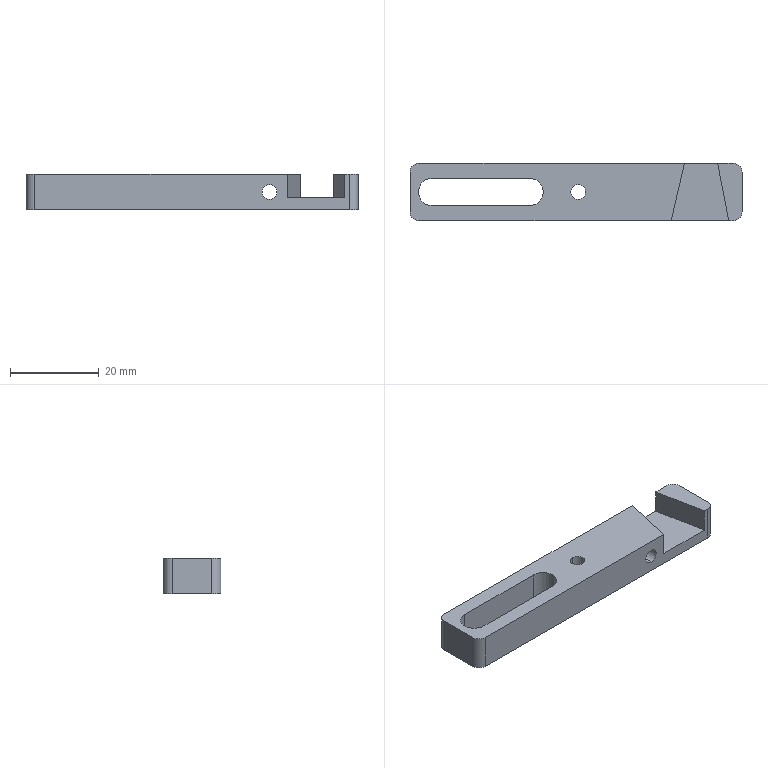Component | SolidWorks | BSH3-02-00ARubberBlankingAssembly2-1_BSH3-02-10FeedBlock2-1 | 1 solid | 22 faces | box 75 x 13 x 8 mm | volume 5554 mm3 | plane 12 | cylinder 10 | commonest cylinder face diameters 3.3 x4 4 x4 6.2 x2
build123d program:
from build123d import *

# Parameters (mm, degrees)
SKETCH1_W         = 13
SKETCH1_H         = 75
EXTRUDE1_DEPTH    = 8
FILLET1_R         = 2
M4_TAPPED_HOLE1_D = 3.3
M4_TAPPED_HOLE2_D = 3.3
EXTRUDE2_DEPTH    = 5.3


with BuildPart() as part:
    # Sketch1 → Extrude1 (new body)
    with BuildSketch(Plane.XY):
        Rectangle(SKETCH1_W, SKETCH1_H)
        with BuildLine():
            Line((3.1, 32.5), (3.1, 10.5))
            ThreePointArc((3.1, 10.5), (0, 7.4), (-3.1, 10.5))
            Line((-3.1, 10.5), (-3.1, 32.5))
            ThreePointArc((-3.1, 32.5), (0, 35.6), (3.1, 32.5))
        make_face(mode=Mode.SUBTRACT)
    extrude(amount=EXTRUDE1_DEPTH)

    # Fillet1
    fillet1_edges = [part.edges().sort_by_distance(p)[0] for p in [
        (6.5, -37.5, 4),
        (-6.5, -37.5, 4),
        (-6.5, 37.5, 4),
        (6.5, 37.5, 4),
    ]]
    fillet(fillet1_edges, radius=FILLET1_R)

    # M4 Tapped Hole1 (through all)
    with Locations(Plane(origin=(0, -0.5, 8), x_dir=(1, 0, 0), z_dir=(0, 0, 1))):
        with Locations((0, 0)):
            Hole(M4_TAPPED_HOLE1_D / 2)

    # M4 Tapped Hole2 (through all)
    with Locations(Plane(origin=(-6.5, -17.5, 4), x_dir=(0, 0, -1), z_dir=(-1, 0, 0))):
        with Locations((0, 0)):
            Hole(M4_TAPPED_HOLE2_D / 2)

    # Sketch4 → Extrude2 (cut)
    with BuildSketch(Plane.XY.offset(8)):
        Polygon((-6.5, -34.5), (6.5, -32), (6.5, -24.5), (-6.5, -21.5), align=None)
    extrude(amount=-EXTRUDE2_DEPTH, mode=Mode.SUBTRACT)


solid = part.part

# Placed as in the assembly
solid = solid.moved(Location((85.129, 20.762, -15.239), (0, 0, 90)))
STEP:
#1=CARTESIAN_POINT('',(4.041,1.073,-0.5074));
#2=VERTEX_POINT('',#1);
#3=CARTESIAN_POINT('',(4.041,1.073,-0.3775));
#4=VERTEX_POINT('',#3);
#5=CARTESIAN_POINT('',(4.041,1.073,-0.4425));
#6=DIRECTION('',(0.,-1.,0.));
#7=DIRECTION('',(0.,0.,1.));
#8=AXIS2_PLACEMENT_3D('',#5,#6,#7);
#9=CIRCLE('',#8,0.06496);
#10=EDGE_CURVE('',#2,#4,#9,.T.);
#11=ORIENTED_EDGE('',*,*,#10,.F.);
#12=CARTESIAN_POINT('',(4.041,0.5615,-0.5074));
#13=VERTEX_POINT('',#12);
#14=CARTESIAN_POINT('',(4.041,0.5615,-0.5074));
#15=DIRECTION('',(0.,-1.,0.));
#16=VECTOR('',#15,39.37);
#17=LINE('',#14,#16);
#18=EDGE_CURVE('',#2,#13,#17,.T.);
#19=ORIENTED_EDGE('',*,*,#18,.T.);
#20=CARTESIAN_POINT('',(4.041,0.5615,-0.3775));
#21=VERTEX_POINT('',#20);
#22=CARTESIAN_POINT('',(4.041,0.5615,-0.4425));
#23=DIRECTION('',(0.,-1.,0.));
#24=DIRECTION('',(0.,0.,1.));
#25=AXIS2_PLACEMENT_3D('',#22,#23,#24);
#26=CIRCLE('',#25,0.06496);
#27=EDGE_CURVE('',#13,#21,#26,.T.);
#28=ORIENTED_EDGE('',*,*,#27,.T.);
#29=CARTESIAN_POINT('',(4.041,0.5615,-0.3775));
#30=DIRECTION('',(0.,-1.,0.));
#31=VECTOR('',#30,39.37);
#32=LINE('',#29,#31);
#33=EDGE_CURVE('',#4,#21,#32,.T.);
#34=ORIENTED_EDGE('',*,*,#33,.F.);
#35=EDGE_LOOP('',(#11,#19,#28,#34));
#36=FACE_OUTER_BOUND('',#35,.T.);
#37=CARTESIAN_POINT('',(4.041,0.5615,-0.4425));
#38=DIRECTION('',(0.,-1.,0.));
#39=DIRECTION('',(0.,0.,1.));
#40=AXIS2_PLACEMENT_3D('',#37,#38,#39);
#41=CYLINDRICAL_SURFACE('',#40,0.06496);
#42=ADVANCED_FACE('',(#36),#41,.F.);
#43=CARTESIAN_POINT('',(3.371,0.7524,-0.6));
#44=VERTEX_POINT('',#43);
#45=CARTESIAN_POINT('',(3.371,0.8823,-0.6));
#46=VERTEX_POINT('',#45);
#47=CARTESIAN_POINT('',(3.371,0.8174,-0.6));
#48=DIRECTION('',(0.,0.,1.));
#49=DIRECTION('',(0.,1.,0.));
#50=AXIS2_PLACEMENT_3D('',#47,#48,#49);
#51=CIRCLE('',#50,0.06496);
#52=EDGE_CURVE('',#44,#46,#51,.T.);
#53=ORIENTED_EDGE('',*,*,#52,.F.);
#54=CARTESIAN_POINT('',(3.371,0.7524,-0.285));
#55=VERTEX_POINT('',#54);
#56=CARTESIAN_POINT('',(3.371,0.7524,-0.285));
#57=DIRECTION('',(0.,0.,1.));
#58=VECTOR('',#57,39.37);
#59=LINE('',#56,#58);
#60=EDGE_CURVE('',#44,#55,#59,.T.);
#61=ORIENTED_EDGE('',*,*,#60,.T.);
#62=CARTESIAN_POINT('',(3.371,0.8823,-0.285));
#63=VERTEX_POINT('',#62);
#64=CARTESIAN_POINT('',(3.371,0.8174,-0.285));
#65=DIRECTION('',(0.,0.,1.));
#66=DIRECTION('',(0.,1.,0.));
#67=AXIS2_PLACEMENT_3D('',#64,#65,#66);
#68=CIRCLE('',#67,0.06496);
#69=EDGE_CURVE('',#55,#63,#68,.T.);
#70=ORIENTED_EDGE('',*,*,#69,.T.);
#71=CARTESIAN_POINT('',(3.371,0.8823,-0.285));
#72=DIRECTION('',(0.,0.,1.));
#73=VECTOR('',#72,39.37);
#74=LINE('',#71,#73);
#75=EDGE_CURVE('',#46,#63,#74,.T.);
#76=ORIENTED_EDGE('',*,*,#75,.F.);
#77=EDGE_LOOP('',(#53,#61,#70,#76));
#78=FACE_OUTER_BOUND('',#77,.T.);
#79=CARTESIAN_POINT('',(3.371,0.8174,-0.285));
#80=DIRECTION('',(0.,0.,1.));
#81=DIRECTION('',(0.,1.,0.));
#82=AXIS2_PLACEMENT_3D('',#79,#80,#81);
#83=CYLINDRICAL_SURFACE('',#82,0.06496);
#84=ADVANCED_FACE('',(#78),#83,.F.);
#85=CARTESIAN_POINT('',(3.371,0.8174,-0.285));
#86=DIRECTION('',(0.,0.,1.));
#87=DIRECTION('',(0.,1.,0.));
#88=AXIS2_PLACEMENT_3D('',#85,#86,#87);
#89=CIRCLE('',#88,0.06496);
#90=EDGE_CURVE('',#63,#55,#89,.T.);
#91=ORIENTED_EDGE('',*,*,#90,.F.);
#92=ORIENTED_EDGE('',*,*,#69,.F.);
#93=EDGE_LOOP('',(#91,#92));
#94=FACE_BOUND('',#93,.T.);
#95=CARTESIAN_POINT('',(2.072,0.9394,-0.285));
#96=VERTEX_POINT('',#95);
#97=CARTESIAN_POINT('',(2.072,0.6953,-0.285));
#98=VERTEX_POINT('',#97);
#99=CARTESIAN_POINT('',(2.072,0.8174,-0.285));
#100=DIRECTION('',(0.,0.,1.));
#101=DIRECTION('',(0.,1.,0.));
#102=AXIS2_PLACEMENT_3D('',#99,#100,#101);
#103=CIRCLE('',#102,0.122);
#104=EDGE_CURVE('',#96,#98,#103,.T.);
#105=ORIENTED_EDGE('',*,*,#104,.F.);
#106=CARTESIAN_POINT('',(2.938,0.9394,-0.285));
#107=VERTEX_POINT('',#106);
#108=CARTESIAN_POINT('',(2.072,0.9394,-0.285));
#109=DIRECTION('',(-1.,-0.,0.));
#110=VECTOR('',#109,39.37);
#111=LINE('',#108,#110);
#112=EDGE_CURVE('',#107,#96,#111,.T.);
#113=ORIENTED_EDGE('',*,*,#112,.F.);
#114=CARTESIAN_POINT('',(2.938,0.6953,-0.285));
#115=VERTEX_POINT('',#114);
#116=CARTESIAN_POINT('',(2.938,0.8174,-0.285));
#117=DIRECTION('',(0.,0.,1.));
#118=DIRECTION('',(0.,1.,0.));
#119=AXIS2_PLACEMENT_3D('',#116,#117,#118);
#120=CIRCLE('',#119,0.122);
#121=EDGE_CURVE('',#115,#107,#120,.T.);
#122=ORIENTED_EDGE('',*,*,#121,.F.);
#123=CARTESIAN_POINT('',(2.072,0.6953,-0.285));
#124=DIRECTION('',(1.,0.,-0.));
#125=VECTOR('',#124,39.37);
#126=LINE('',#123,#125);
#127=EDGE_CURVE('',#98,#115,#126,.T.);
#128=ORIENTED_EDGE('',*,*,#127,.F.);
#129=EDGE_LOOP('',(#105,#113,#122,#128));
#130=FACE_BOUND('',#129,.T.);
#131=CARTESIAN_POINT('',(1.954,0.5615,-0.285));
#132=VERTEX_POINT('',#131);
#133=CARTESIAN_POINT('',(4.198,0.5615,-0.285));
#134=VERTEX_POINT('',#133);
#135=CARTESIAN_POINT('',(4.828,0.5615,-0.285));
#136=DIRECTION('',(1.,0.,-0.));
#137=VECTOR('',#136,39.37);
#138=LINE('',#135,#137);
#139=EDGE_CURVE('',#132,#134,#138,.T.);
#140=ORIENTED_EDGE('',*,*,#139,.T.);
#141=CARTESIAN_POINT('',(4.316,1.073,-0.285));
#142=VERTEX_POINT('',#141);
#143=CARTESIAN_POINT('',(4.316,1.073,-0.285));
#144=DIRECTION('',(-0.2249,-0.9744,0.));
#145=VECTOR('',#144,39.37);
#146=LINE('',#143,#145);
#147=EDGE_CURVE('',#142,#134,#146,.T.);
#148=ORIENTED_EDGE('',*,*,#147,.F.);
#149=CARTESIAN_POINT('',(1.954,1.073,-0.285));
#150=VERTEX_POINT('',#149);
#151=CARTESIAN_POINT('',(4.828,1.073,-0.285));
#152=DIRECTION('',(-1.,-0.,0.));
#153=VECTOR('',#152,39.37);
#154=LINE('',#151,#153);
#155=EDGE_CURVE('',#142,#150,#154,.T.);
#156=ORIENTED_EDGE('',*,*,#155,.T.);
#157=CARTESIAN_POINT('',(1.875,0.9946,-0.285));
#158=VERTEX_POINT('',#157);
#159=CARTESIAN_POINT('',(1.954,0.9946,-0.285));
#160=DIRECTION('',(0.,0.,1.));
#161=DIRECTION('',(0.,-1.,0.));
#162=AXIS2_PLACEMENT_3D('',#159,#160,#161);
#163=CIRCLE('',#162,0.07874);
#164=EDGE_CURVE('',#150,#158,#163,.T.);
#165=ORIENTED_EDGE('',*,*,#164,.T.);
#166=CARTESIAN_POINT('',(1.875,0.6402,-0.285));
#167=VERTEX_POINT('',#166);
#168=CARTESIAN_POINT('',(1.875,0.5615,-0.285));
#169=DIRECTION('',(0.,-1.,0.));
#170=VECTOR('',#169,39.37);
#171=LINE('',#168,#170);
#172=EDGE_CURVE('',#158,#167,#171,.T.);
#173=ORIENTED_EDGE('',*,*,#172,.T.);
#174=CARTESIAN_POINT('',(1.954,0.6402,-0.285));
#175=DIRECTION('',(0.,0.,1.));
#176=DIRECTION('',(0.,-1.,0.));
#177=AXIS2_PLACEMENT_3D('',#174,#175,#176);
#178=CIRCLE('',#177,0.07874);
#179=EDGE_CURVE('',#167,#132,#178,.T.);
#180=ORIENTED_EDGE('',*,*,#179,.T.);
#181=EDGE_LOOP('',(#140,#148,#156,#165,#173,#180));
#182=FACE_OUTER_BOUND('',#181,.T.);
#183=CARTESIAN_POINT('',(1.875,1.073,-0.285));
#184=DIRECTION('',(-0.,-0.,-1.));
#185=DIRECTION('',(0.,-1.,0.));
#186=AXIS2_PLACEMENT_3D('',#183,#184,#185);
#187=PLANE('',#186);
#188=ADVANCED_FACE('',(#94,#130,#182),#187,.F.);
#189=CARTESIAN_POINT('',(4.749,1.073,-0.285));
#190=VERTEX_POINT('',#189);
#191=CARTESIAN_POINT('',(4.611,1.073,-0.285));
#192=VERTEX_POINT('',#191);
#193=CARTESIAN_POINT('',(4.828,1.073,-0.285));
#194=DIRECTION('',(-1.,-0.,0.));
#195=VECTOR('',#194,39.37);
#196=LINE('',#193,#195);
#197=EDGE_CURVE('',#190,#192,#196,.T.);
#198=ORIENTED_EDGE('',*,*,#197,.T.);
#199=CARTESIAN_POINT('',(4.71,0.5615,-0.285));
#200=VERTEX_POINT('',#199);
#201=CARTESIAN_POINT('',(4.71,0.5615,-0.285));
#202=DIRECTION('',(-0.1888,0.982,-0.));
#203=VECTOR('',#202,39.37);
#204=LINE('',#201,#203);
#205=EDGE_CURVE('',#200,#192,#204,.T.);
#206=ORIENTED_EDGE('',*,*,#205,.F.);
#207=CARTESIAN_POINT('',(4.749,0.5615,-0.285));
#208=VERTEX_POINT('',#207);
#209=CARTESIAN_POINT('',(4.828,0.5615,-0.285));
#210=DIRECTION('',(1.,0.,-0.));
#211=VECTOR('',#210,39.37);
#212=LINE('',#209,#211);
#213=EDGE_CURVE('',#200,#208,#212,.T.);
#214=ORIENTED_EDGE('',*,*,#213,.T.);
#215=CARTESIAN_POINT('',(4.828,0.6402,-0.285));
#216=VERTEX_POINT('',#215);
#217=CARTESIAN_POINT('',(4.749,0.6402,-0.285));
#218=DIRECTION('',(0.,0.,1.));
#219=DIRECTION('',(0.,-1.,0.));
#220=AXIS2_PLACEMENT_3D('',#217,#218,#219);
#221=CIRCLE('',#220,0.07874);
#222=EDGE_CURVE('',#208,#216,#221,.T.);
#223=ORIENTED_EDGE('',*,*,#222,.T.);
#224=CARTESIAN_POINT('',(4.828,0.9946,-0.285));
#225=VERTEX_POINT('',#224);
#226=CARTESIAN_POINT('',(4.828,0.5615,-0.285));
#227=DIRECTION('',(-0.,1.,-0.));
#228=VECTOR('',#227,39.37);
#229=LINE('',#226,#228);
#230=EDGE_CURVE('',#216,#225,#229,.T.);
#231=ORIENTED_EDGE('',*,*,#230,.T.);
#232=CARTESIAN_POINT('',(4.749,0.9946,-0.285));
#233=DIRECTION('',(0.,0.,1.));
#234=DIRECTION('',(0.,-1.,0.));
#235=AXIS2_PLACEMENT_3D('',#232,#233,#234);
#236=CIRCLE('',#235,0.07874);
#237=EDGE_CURVE('',#225,#190,#236,.T.);
#238=ORIENTED_EDGE('',*,*,#237,.T.);
#239=EDGE_LOOP('',(#198,#206,#214,#223,#231,#238));
#240=FACE_OUTER_BOUND('',#239,.T.);
#241=CARTESIAN_POINT('',(1.875,1.073,-0.285));
#242=DIRECTION('',(-0.,-0.,-1.));
#243=DIRECTION('',(0.,-1.,0.));
#244=AXIS2_PLACEMENT_3D('',#241,#242,#243);
#245=PLANE('',#244);
#246=ADVANCED_FACE('',(#240),#245,.F.);
#247=CARTESIAN_POINT('',(2.938,0.9394,-0.6));
#248=VERTEX_POINT('',#247);
#249=CARTESIAN_POINT('',(2.072,0.9394,-0.6));
#250=VERTEX_POINT('',#249);
#251=CARTESIAN_POINT('',(2.072,0.9394,-0.6));
#252=DIRECTION('',(-1.,-0.,0.));
#253=VECTOR('',#252,39.37);
#254=LINE('',#251,#253);
#255=EDGE_CURVE('',#248,#250,#254,.T.);
#256=ORIENTED_EDGE('',*,*,#255,.T.);
#257=CARTESIAN_POINT('',(2.072,0.6953,-0.6));
#258=VERTEX_POINT('',#257);
#259=CARTESIAN_POINT('',(2.072,0.8174,-0.6));
#260=DIRECTION('',(0.,0.,1.));
#261=DIRECTION('',(0.,1.,0.));
#262=AXIS2_PLACEMENT_3D('',#259,#260,#261);
#263=CIRCLE('',#262,0.122);
#264=EDGE_CURVE('',#250,#258,#263,.T.);
#265=ORIENTED_EDGE('',*,*,#264,.T.);
#266=CARTESIAN_POINT('',(2.938,0.6953,-0.6));
#267=VERTEX_POINT('',#266);
#268=CARTESIAN_POINT('',(2.072,0.6953,-0.6));
#269=DIRECTION('',(1.,0.,-0.));
#270=VECTOR('',#269,39.37);
#271=LINE('',#268,#270);
#272=EDGE_CURVE('',#258,#267,#271,.T.);
#273=ORIENTED_EDGE('',*,*,#272,.T.);
#274=CARTESIAN_POINT('',(2.938,0.8174,-0.6));
#275=DIRECTION('',(0.,0.,1.));
#276=DIRECTION('',(0.,1.,0.));
#277=AXIS2_PLACEMENT_3D('',#274,#275,#276);
#278=CIRCLE('',#277,0.122);
#279=EDGE_CURVE('',#267,#248,#278,.T.);
#280=ORIENTED_EDGE('',*,*,#279,.T.);
#281=EDGE_LOOP('',(#256,#265,#273,#280));
#282=FACE_BOUND('',#281,.T.);
#283=CARTESIAN_POINT('',(4.749,1.073,-0.6));
#284=VERTEX_POINT('',#283);
#285=CARTESIAN_POINT('',(1.954,1.073,-0.6));
#286=VERTEX_POINT('',#285);
#287=CARTESIAN_POINT('',(4.828,1.073,-0.6));
#288=DIRECTION('',(-1.,-0.,0.));
#289=VECTOR('',#288,39.37);
#290=LINE('',#287,#289);
#291=EDGE_CURVE('',#284,#286,#290,.T.);
#292=ORIENTED_EDGE('',*,*,#291,.F.);
#293=CARTESIAN_POINT('',(4.828,0.9946,-0.6));
#294=VERTEX_POINT('',#293);
#295=CARTESIAN_POINT('',(4.749,0.9946,-0.6));
#296=DIRECTION('',(-0.,-0.,-1.));
#297=DIRECTION('',(0.,-1.,0.));
#298=AXIS2_PLACEMENT_3D('',#295,#296,#297);
#299=CIRCLE('',#298,0.07874);
#300=EDGE_CURVE('',#284,#294,#299,.T.);
#301=ORIENTED_EDGE('',*,*,#300,.T.);
#302=CARTESIAN_POINT('',(4.828,0.6402,-0.6));
#303=VERTEX_POINT('',#302);
#304=CARTESIAN_POINT('',(4.828,0.5615,-0.6));
#305=DIRECTION('',(-0.,1.,-0.));
#306=VECTOR('',#305,39.37);
#307=LINE('',#304,#306);
#308=EDGE_CURVE('',#303,#294,#307,.T.);
#309=ORIENTED_EDGE('',*,*,#308,.F.);
#310=CARTESIAN_POINT('',(4.749,0.5615,-0.6));
#311=VERTEX_POINT('',#310);
#312=CARTESIAN_POINT('',(4.749,0.6402,-0.6));
#313=DIRECTION('',(-0.,-0.,-1.));
#314=DIRECTION('',(0.,-1.,0.));
#315=AXIS2_PLACEMENT_3D('',#312,#313,#314);
#316=CIRCLE('',#315,0.07874);
#317=EDGE_CURVE('',#303,#311,#316,.T.);
#318=ORIENTED_EDGE('',*,*,#317,.T.);
#319=CARTESIAN_POINT('',(1.954,0.5615,-0.6));
#320=VERTEX_POINT('',#319);
#321=CARTESIAN_POINT('',(4.828,0.5615,-0.6));
#322=DIRECTION('',(1.,0.,-0.));
#323=VECTOR('',#322,39.37);
#324=LINE('',#321,#323);
#325=EDGE_CURVE('',#320,#311,#324,.T.);
#326=ORIENTED_EDGE('',*,*,#325,.F.);
#327=CARTESIAN_POINT('',(1.875,0.6402,-0.6));
#328=VERTEX_POINT('',#327);
#329=CARTESIAN_POINT('',(1.954,0.6402,-0.6));
#330=DIRECTION('',(-0.,-0.,-1.));
#331=DIRECTION('',(0.,-1.,0.));
#332=AXIS2_PLACEMENT_3D('',#329,#330,#331);
#333=CIRCLE('',#332,0.07874);
#334=EDGE_CURVE('',#320,#328,#333,.T.);
#335=ORIENTED_EDGE('',*,*,#334,.T.);
#336=CARTESIAN_POINT('',(1.875,0.9946,-0.6));
#337=VERTEX_POINT('',#336);
#338=CARTESIAN_POINT('',(1.875,0.5615,-0.6));
#339=DIRECTION('',(0.,-1.,0.));
#340=VECTOR('',#339,39.37);
#341=LINE('',#338,#340);
#342=EDGE_CURVE('',#337,#328,#341,.T.);
#343=ORIENTED_EDGE('',*,*,#342,.F.);
#344=CARTESIAN_POINT('',(1.954,0.9946,-0.6));
#345=DIRECTION('',(-0.,-0.,-1.));
#346=DIRECTION('',(0.,-1.,0.));
#347=AXIS2_PLACEMENT_3D('',#344,#345,#346);
#348=CIRCLE('',#347,0.07874);
#349=EDGE_CURVE('',#337,#286,#348,.T.);
#350=ORIENTED_EDGE('',*,*,#349,.T.);
#351=EDGE_LOOP('',(#292,#301,#309,#318,#326,#335,#343,#350));
#352=FACE_OUTER_BOUND('',#351,.T.);
#353=CARTESIAN_POINT('',(3.371,0.8174,-0.6));
#354=DIRECTION('',(0.,0.,1.));
#355=DIRECTION('',(0.,1.,0.));
#356=AXIS2_PLACEMENT_3D('',#353,#354,#355);
#357=CIRCLE('',#356,0.06496);
#358=EDGE_CURVE('',#46,#44,#357,.T.);
#359=ORIENTED_EDGE('',*,*,#358,.T.);
#360=ORIENTED_EDGE('',*,*,#52,.T.);
#361=EDGE_LOOP('',(#359,#360));
#362=FACE_BOUND('',#361,.T.);
#363=CARTESIAN_POINT('',(1.875,1.073,-0.6));
#364=DIRECTION('',(-0.,-0.,-1.));
#365=DIRECTION('',(0.,-1.,0.));
#366=AXIS2_PLACEMENT_3D('',#363,#364,#365);
#367=PLANE('',#366);
#368=ADVANCED_FACE('',(#282,#352,#362),#367,.T.);
#369=ORIENTED_EDGE('',*,*,#155,.F.);
#370=CARTESIAN_POINT('',(4.316,1.073,-0.4937));
#371=VERTEX_POINT('',#370);
#372=CARTESIAN_POINT('',(4.316,1.073,-0.4937));
#373=DIRECTION('',(0.,0.,1.));
#374=VECTOR('',#373,39.37);
#375=LINE('',#372,#374);
#376=EDGE_CURVE('',#371,#142,#375,.T.);
#377=ORIENTED_EDGE('',*,*,#376,.F.);
#378=CARTESIAN_POINT('',(4.611,1.073,-0.4937));
#379=VERTEX_POINT('',#378);
#380=CARTESIAN_POINT('',(4.611,1.073,-0.4937));
#381=DIRECTION('',(-1.,-0.,0.));
#382=VECTOR('',#381,39.37);
#383=LINE('',#380,#382);
#384=EDGE_CURVE('',#379,#371,#383,.T.);
#385=ORIENTED_EDGE('',*,*,#384,.F.);
#386=CARTESIAN_POINT('',(4.611,1.073,-0.4937));
#387=DIRECTION('',(0.,0.,1.));
#388=VECTOR('',#387,39.37);
#389=LINE('',#386,#388);
#390=EDGE_CURVE('',#379,#192,#389,.T.);
#391=ORIENTED_EDGE('',*,*,#390,.T.);
#392=ORIENTED_EDGE('',*,*,#197,.F.);
#393=CARTESIAN_POINT('',(4.749,1.073,-0.285));
#394=DIRECTION('',(-0.,-0.,-1.));
#395=VECTOR('',#394,39.37);
#396=LINE('',#393,#395);
#397=EDGE_CURVE('',#190,#284,#396,.T.);
#398=ORIENTED_EDGE('',*,*,#397,.T.);
#399=ORIENTED_EDGE('',*,*,#291,.T.);
#400=CARTESIAN_POINT('',(1.954,1.073,-0.285));
#401=DIRECTION('',(0.,0.,1.));
#402=VECTOR('',#401,39.37);
#403=LINE('',#400,#402);
#404=EDGE_CURVE('',#286,#150,#403,.T.);
#405=ORIENTED_EDGE('',*,*,#404,.T.);
#406=EDGE_LOOP('',(#369,#377,#385,#391,#392,#398,#399,#405));
#407=FACE_OUTER_BOUND('',#406,.T.);
#408=CARTESIAN_POINT('',(4.041,1.073,-0.4425));
#409=DIRECTION('',(0.,-1.,0.));
#410=DIRECTION('',(0.,0.,1.));
#411=AXIS2_PLACEMENT_3D('',#408,#409,#410);
#412=CIRCLE('',#411,0.06496);
#413=EDGE_CURVE('',#4,#2,#412,.T.);
#414=ORIENTED_EDGE('',*,*,#413,.T.);
#415=ORIENTED_EDGE('',*,*,#10,.T.);
#416=EDGE_LOOP('',(#414,#415));
#417=FACE_BOUND('',#416,.T.);
#418=CARTESIAN_POINT('',(4.828,1.073,-0.285));
#419=DIRECTION('',(0.,-1.,0.));
#420=DIRECTION('',(0.,0.,1.));
#421=AXIS2_PLACEMENT_3D('',#418,#419,#420);
#422=PLANE('',#421);
#423=ADVANCED_FACE('',(#407,#417),#422,.F.);
#424=ORIENTED_EDGE('',*,*,#342,.T.);
#425=CARTESIAN_POINT('',(1.875,0.6402,-0.285));
#426=DIRECTION('',(0.,0.,1.));
#427=VECTOR('',#426,39.37);
#428=LINE('',#425,#427);
#429=EDGE_CURVE('',#328,#167,#428,.T.);
#430=ORIENTED_EDGE('',*,*,#429,.T.);
#431=ORIENTED_EDGE('',*,*,#172,.F.);
#432=CARTESIAN_POINT('',(1.875,0.9946,-0.285));
#433=DIRECTION('',(-0.,-0.,-1.));
#434=VECTOR('',#433,39.37);
#435=LINE('',#432,#434);
#436=EDGE_CURVE('',#158,#337,#435,.T.);
#437=ORIENTED_EDGE('',*,*,#436,.T.);
#438=EDGE_LOOP('',(#424,#430,#431,#437));
#439=FACE_OUTER_BOUND('',#438,.T.);
#440=CARTESIAN_POINT('',(1.875,0.5615,-0.285));
#441=DIRECTION('',(1.,0.,-0.));
#442=DIRECTION('',(-0.,-0.,-1.));
#443=AXIS2_PLACEMENT_3D('',#440,#441,#442);
#444=PLANE('',#443);
#445=ADVANCED_FACE('',(#439),#444,.F.);
#446=CARTESIAN_POINT('',(4.041,0.5615,-0.4425));
#447=DIRECTION('',(0.,-1.,0.));
#448=DIRECTION('',(0.,0.,1.));
#449=AXIS2_PLACEMENT_3D('',#446,#447,#448);
#450=CIRCLE('',#449,0.06496);
#451=EDGE_CURVE('',#21,#13,#450,.T.);
#452=ORIENTED_EDGE('',*,*,#451,.F.);
#453=ORIENTED_EDGE('',*,*,#27,.F.);
#454=EDGE_LOOP('',(#452,#453));
#455=FACE_BOUND('',#454,.T.);
#456=CARTESIAN_POINT('',(4.198,0.5615,-0.4937));
#457=VERTEX_POINT('',#456);
#458=CARTESIAN_POINT('',(4.71,0.5615,-0.4937));
#459=VERTEX_POINT('',#458);
#460=CARTESIAN_POINT('',(4.198,0.5615,-0.4937));
#461=DIRECTION('',(1.,0.,-0.));
#462=VECTOR('',#461,39.37);
#463=LINE('',#460,#462);
#464=EDGE_CURVE('',#457,#459,#463,.T.);
#465=ORIENTED_EDGE('',*,*,#464,.F.);
#466=CARTESIAN_POINT('',(4.198,0.5615,-0.4937));
#467=DIRECTION('',(0.,0.,1.));
#468=VECTOR('',#467,39.37);
#469=LINE('',#466,#468);
#470=EDGE_CURVE('',#457,#134,#469,.T.);
#471=ORIENTED_EDGE('',*,*,#470,.T.);
#472=ORIENTED_EDGE('',*,*,#139,.F.);
#473=CARTESIAN_POINT('',(1.954,0.5615,-0.285));
#474=DIRECTION('',(-0.,-0.,-1.));
#475=VECTOR('',#474,39.37);
#476=LINE('',#473,#475);
#477=EDGE_CURVE('',#132,#320,#476,.T.);
#478=ORIENTED_EDGE('',*,*,#477,.T.);
#479=ORIENTED_EDGE('',*,*,#325,.T.);
#480=CARTESIAN_POINT('',(4.749,0.5615,-0.285));
#481=DIRECTION('',(0.,0.,1.));
#482=VECTOR('',#481,39.37);
#483=LINE('',#480,#482);
#484=EDGE_CURVE('',#311,#208,#483,.T.);
#485=ORIENTED_EDGE('',*,*,#484,.T.);
#486=ORIENTED_EDGE('',*,*,#213,.F.);
#487=CARTESIAN_POINT('',(4.71,0.5615,-0.4937));
#488=DIRECTION('',(0.,0.,1.));
#489=VECTOR('',#488,39.37);
#490=LINE('',#487,#489);
#491=EDGE_CURVE('',#459,#200,#490,.T.);
#492=ORIENTED_EDGE('',*,*,#491,.F.);
#493=EDGE_LOOP('',(#465,#471,#472,#478,#479,#485,#486,#492));
#494=FACE_OUTER_BOUND('',#493,.T.);
#495=CARTESIAN_POINT('',(4.828,0.5615,-0.285));
#496=DIRECTION('',(-0.,1.,-0.));
#497=DIRECTION('',(-0.,-0.,-1.));
#498=AXIS2_PLACEMENT_3D('',#495,#496,#497);
#499=PLANE('',#498);
#500=ADVANCED_FACE('',(#455,#494),#499,.F.);
#501=ORIENTED_EDGE('',*,*,#308,.T.);
#502=CARTESIAN_POINT('',(4.828,0.9946,-0.285));
#503=DIRECTION('',(0.,0.,1.));
#504=VECTOR('',#503,39.37);
#505=LINE('',#502,#504);
#506=EDGE_CURVE('',#294,#225,#505,.T.);
#507=ORIENTED_EDGE('',*,*,#506,.T.);
#508=ORIENTED_EDGE('',*,*,#230,.F.);
#509=CARTESIAN_POINT('',(4.828,0.6402,-0.285));
#510=DIRECTION('',(-0.,-0.,-1.));
#511=VECTOR('',#510,39.37);
#512=LINE('',#509,#511);
#513=EDGE_CURVE('',#216,#303,#512,.T.);
#514=ORIENTED_EDGE('',*,*,#513,.T.);
#515=EDGE_LOOP('',(#501,#507,#508,#514));
#516=FACE_OUTER_BOUND('',#515,.T.);
#517=CARTESIAN_POINT('',(4.828,0.5615,-0.285));
#518=DIRECTION('',(-1.,-0.,0.));
#519=DIRECTION('',(0.,0.,1.));
#520=AXIS2_PLACEMENT_3D('',#517,#518,#519);
#521=PLANE('',#520);
#522=ADVANCED_FACE('',(#516),#521,.F.);
#523=ORIENTED_EDGE('',*,*,#264,.F.);
#524=CARTESIAN_POINT('',(2.072,0.9394,-0.285));
#525=DIRECTION('',(-0.,-0.,-1.));
#526=VECTOR('',#525,39.37);
#527=LINE('',#524,#526);
#528=EDGE_CURVE('',#96,#250,#527,.T.);
#529=ORIENTED_EDGE('',*,*,#528,.F.);
#530=ORIENTED_EDGE('',*,*,#104,.T.);
#531=CARTESIAN_POINT('',(2.072,0.6953,-0.285));
#532=DIRECTION('',(-0.,-0.,-1.));
#533=VECTOR('',#532,39.37);
#534=LINE('',#531,#533);
#535=EDGE_CURVE('',#98,#258,#534,.T.);
#536=ORIENTED_EDGE('',*,*,#535,.T.);
#537=EDGE_LOOP('',(#523,#529,#530,#536));
#538=FACE_OUTER_BOUND('',#537,.T.);
#539=CARTESIAN_POINT('',(2.072,0.8174,-0.285));
#540=DIRECTION('',(-0.,-0.,-1.));
#541=DIRECTION('',(0.,-1.,0.));
#542=AXIS2_PLACEMENT_3D('',#539,#540,#541);
#543=CYLINDRICAL_SURFACE('',#542,0.122);
#544=ADVANCED_FACE('',(#538),#543,.F.);
#545=ORIENTED_EDGE('',*,*,#272,.F.);
#546=ORIENTED_EDGE('',*,*,#535,.F.);
#547=ORIENTED_EDGE('',*,*,#127,.T.);
#548=CARTESIAN_POINT('',(2.938,0.6953,-0.285));
#549=DIRECTION('',(-0.,-0.,-1.));
#550=VECTOR('',#549,39.37);
#551=LINE('',#548,#550);
#552=EDGE_CURVE('',#115,#267,#551,.T.);
#553=ORIENTED_EDGE('',*,*,#552,.T.);
#554=EDGE_LOOP('',(#545,#546,#547,#553));
#555=FACE_OUTER_BOUND('',#554,.T.);
#556=CARTESIAN_POINT('',(2.072,0.6953,-0.285));
#557=DIRECTION('',(-0.,1.,-0.));
#558=DIRECTION('',(-1.,-0.,0.));
#559=AXIS2_PLACEMENT_3D('',#556,#557,#558);
#560=PLANE('',#559);
#561=ADVANCED_FACE('',(#555),#560,.T.);
#562=ORIENTED_EDGE('',*,*,#279,.F.);
#563=ORIENTED_EDGE('',*,*,#552,.F.);
#564=ORIENTED_EDGE('',*,*,#121,.T.);
#565=CARTESIAN_POINT('',(2.938,0.9394,-0.285));
#566=DIRECTION('',(-0.,-0.,-1.));
#567=VECTOR('',#566,39.37);
#568=LINE('',#565,#567);
#569=EDGE_CURVE('',#107,#248,#568,.T.);
#570=ORIENTED_EDGE('',*,*,#569,.T.);
#571=EDGE_LOOP('',(#562,#563,#564,#570));
#572=FACE_OUTER_BOUND('',#571,.T.);
#573=CARTESIAN_POINT('',(2.938,0.8174,-0.285));
#574=DIRECTION('',(-0.,-0.,-1.));
#575=DIRECTION('',(0.,-1.,0.));
#576=AXIS2_PLACEMENT_3D('',#573,#574,#575);
#577=CYLINDRICAL_SURFACE('',#576,0.122);
#578=ADVANCED_FACE('',(#572),#577,.F.);
#579=ORIENTED_EDGE('',*,*,#255,.F.);
#580=ORIENTED_EDGE('',*,*,#569,.F.);
#581=ORIENTED_EDGE('',*,*,#112,.T.);
#582=ORIENTED_EDGE('',*,*,#528,.T.);
#583=EDGE_LOOP('',(#579,#580,#581,#582));
#584=FACE_OUTER_BOUND('',#583,.T.);
#585=CARTESIAN_POINT('',(2.072,0.9394,-0.285));
#586=DIRECTION('',(0.,-1.,0.));
#587=DIRECTION('',(1.,0.,-0.));
#588=AXIS2_PLACEMENT_3D('',#585,#586,#587);
#589=PLANE('',#588);
#590=ADVANCED_FACE('',(#584),#589,.T.);
#591=ORIENTED_EDGE('',*,*,#237,.F.);
#592=ORIENTED_EDGE('',*,*,#506,.F.);
#593=ORIENTED_EDGE('',*,*,#300,.F.);
#594=ORIENTED_EDGE('',*,*,#397,.F.);
#595=EDGE_LOOP('',(#591,#592,#593,#594));
#596=FACE_OUTER_BOUND('',#595,.T.);
#597=CARTESIAN_POINT('',(4.749,0.9946,-0.285));
#598=DIRECTION('',(-0.,-0.,-1.));
#599=DIRECTION('',(0.,-1.,0.));
#600=AXIS2_PLACEMENT_3D('',#597,#598,#599);
#601=CYLINDRICAL_SURFACE('',#600,0.07874);
#602=ADVANCED_FACE('',(#596),#601,.T.);
#603=ORIENTED_EDGE('',*,*,#222,.F.);
#604=ORIENTED_EDGE('',*,*,#484,.F.);
#605=ORIENTED_EDGE('',*,*,#317,.F.);
#606=ORIENTED_EDGE('',*,*,#513,.F.);
#607=EDGE_LOOP('',(#603,#604,#605,#606));
#608=FACE_OUTER_BOUND('',#607,.T.);
#609=CARTESIAN_POINT('',(4.749,0.6402,-0.285));
#610=DIRECTION('',(-0.,-0.,-1.));
#611=DIRECTION('',(0.,-1.,0.));
#612=AXIS2_PLACEMENT_3D('',#609,#610,#611);
#613=CYLINDRICAL_SURFACE('',#612,0.07874);
#614=ADVANCED_FACE('',(#608),#613,.T.);
#615=ORIENTED_EDGE('',*,*,#179,.F.);
#616=ORIENTED_EDGE('',*,*,#429,.F.);
#617=ORIENTED_EDGE('',*,*,#334,.F.);
#618=ORIENTED_EDGE('',*,*,#477,.F.);
#619=EDGE_LOOP('',(#615,#616,#617,#618));
#620=FACE_OUTER_BOUND('',#619,.T.);
#621=CARTESIAN_POINT('',(1.954,0.6402,-0.285));
#622=DIRECTION('',(-0.,-0.,-1.));
#623=DIRECTION('',(0.,-1.,0.));
#624=AXIS2_PLACEMENT_3D('',#621,#622,#623);
#625=CYLINDRICAL_SURFACE('',#624,0.07874);
#626=ADVANCED_FACE('',(#620),#625,.T.);
#627=ORIENTED_EDGE('',*,*,#164,.F.);
#628=ORIENTED_EDGE('',*,*,#404,.F.);
#629=ORIENTED_EDGE('',*,*,#349,.F.);
#630=ORIENTED_EDGE('',*,*,#436,.F.);
#631=EDGE_LOOP('',(#627,#628,#629,#630));
#632=FACE_OUTER_BOUND('',#631,.T.);
#633=CARTESIAN_POINT('',(1.954,0.9946,-0.285));
#634=DIRECTION('',(-0.,-0.,-1.));
#635=DIRECTION('',(0.,-1.,0.));
#636=AXIS2_PLACEMENT_3D('',#633,#634,#635);
#637=CYLINDRICAL_SURFACE('',#636,0.07874);
#638=ADVANCED_FACE('',(#632),#637,.T.);
#639=ORIENTED_EDGE('',*,*,#60,.F.);
#640=ORIENTED_EDGE('',*,*,#358,.F.);
#641=ORIENTED_EDGE('',*,*,#75,.T.);
#642=ORIENTED_EDGE('',*,*,#90,.T.);
#643=EDGE_LOOP('',(#639,#640,#641,#642));
#644=FACE_OUTER_BOUND('',#643,.T.);
#645=CARTESIAN_POINT('',(3.371,0.8174,-0.285));
#646=DIRECTION('',(0.,0.,1.));
#647=DIRECTION('',(0.,1.,0.));
#648=AXIS2_PLACEMENT_3D('',#645,#646,#647);
#649=CYLINDRICAL_SURFACE('',#648,0.06496);
#650=ADVANCED_FACE('',(#644),#649,.F.);
#651=ORIENTED_EDGE('',*,*,#18,.F.);
#652=ORIENTED_EDGE('',*,*,#413,.F.);
#653=ORIENTED_EDGE('',*,*,#33,.T.);
#654=ORIENTED_EDGE('',*,*,#451,.T.);
#655=EDGE_LOOP('',(#651,#652,#653,#654));
#656=FACE_OUTER_BOUND('',#655,.T.);
#657=CARTESIAN_POINT('',(4.041,0.5615,-0.4425));
#658=DIRECTION('',(0.,-1.,0.));
#659=DIRECTION('',(0.,0.,1.));
#660=AXIS2_PLACEMENT_3D('',#657,#658,#659);
#661=CYLINDRICAL_SURFACE('',#660,0.06496);
#662=ADVANCED_FACE('',(#656),#661,.F.);
#663=ORIENTED_EDGE('',*,*,#147,.T.);
#664=ORIENTED_EDGE('',*,*,#470,.F.);
#665=CARTESIAN_POINT('',(4.316,1.073,-0.4937));
#666=DIRECTION('',(-0.2249,-0.9744,0.));
#667=VECTOR('',#666,39.37);
#668=LINE('',#665,#667);
#669=EDGE_CURVE('',#371,#457,#668,.T.);
#670=ORIENTED_EDGE('',*,*,#669,.F.);
#671=ORIENTED_EDGE('',*,*,#376,.T.);
#672=EDGE_LOOP('',(#663,#664,#670,#671));
#673=FACE_OUTER_BOUND('',#672,.T.);
#674=CARTESIAN_POINT('',(4.316,1.073,-0.4937));
#675=DIRECTION('',(-0.9744,0.2249,0.));
#676=DIRECTION('',(-0.2249,-0.9744,0.));
#677=AXIS2_PLACEMENT_3D('',#674,#675,#676);
#678=PLANE('',#677);
#679=ADVANCED_FACE('',(#673),#678,.F.);
#680=ORIENTED_EDGE('',*,*,#205,.T.);
#681=ORIENTED_EDGE('',*,*,#390,.F.);
#682=CARTESIAN_POINT('',(4.71,0.5615,-0.4937));
#683=DIRECTION('',(-0.1888,0.982,-0.));
#684=VECTOR('',#683,39.37);
#685=LINE('',#682,#684);
#686=EDGE_CURVE('',#459,#379,#685,.T.);
#687=ORIENTED_EDGE('',*,*,#686,.F.);
#688=ORIENTED_EDGE('',*,*,#491,.T.);
#689=EDGE_LOOP('',(#680,#681,#687,#688));
#690=FACE_OUTER_BOUND('',#689,.T.);
#691=CARTESIAN_POINT('',(4.71,0.5615,-0.4937));
#692=DIRECTION('',(0.982,0.1888,-0.));
#693=DIRECTION('',(-0.1888,0.982,-0.));
#694=AXIS2_PLACEMENT_3D('',#691,#692,#693);
#695=PLANE('',#694);
#696=ADVANCED_FACE('',(#690),#695,.F.);
#697=ORIENTED_EDGE('',*,*,#464,.T.);
#698=ORIENTED_EDGE('',*,*,#686,.T.);
#699=ORIENTED_EDGE('',*,*,#384,.T.);
#700=ORIENTED_EDGE('',*,*,#669,.T.);
#701=EDGE_LOOP('',(#697,#698,#699,#700));
#702=FACE_OUTER_BOUND('',#701,.T.);
#703=CARTESIAN_POINT('',(4.71,0.5615,-0.4937));
#704=DIRECTION('',(0.,0.,1.));
#705=DIRECTION('',(-0.,1.,-0.));
#706=AXIS2_PLACEMENT_3D('',#703,#704,#705);
#707=PLANE('',#706);
#708=ADVANCED_FACE('',(#702),#707,.T.);
#709=CLOSED_SHELL('',(#42,#84,#188,#246,#368,#423,#445,#500,#522,#544,#561,#578,#590,#602,#614,#626,#638,#650,#662,#679,#696,#708));
#710=MANIFOLD_SOLID_BREP('',#709);
#711=CARTESIAN_POINT('',(0.,0.,0.));
#712=DIRECTION('',(0.,0.,1.));
#713=DIRECTION('',(1.,0.,0.));
#714=AXIS2_PLACEMENT_3D('',#711,#712,#713);
#715=(LENGTH_UNIT()NAMED_UNIT(*)SI_UNIT($,.METRE.));
#716=LENGTH_MEASURE_WITH_UNIT(LENGTH_MEASURE(0.0254),#715);
#717=DIMENSIONAL_EXPONENTS(1.,0.,0.,0.,0.,0.,0.);
#718=(CONVERSION_BASED_UNIT('',#716)LENGTH_UNIT()NAMED_UNIT(#717));
#719=UNCERTAINTY_MEASURE_WITH_UNIT(LENGTH_MEASURE(0.00001),#718,'','');
#720=(NAMED_UNIT(*)PLANE_ANGLE_UNIT()SI_UNIT($,.RADIAN.));
#721=(NAMED_UNIT(*)SI_UNIT($,.STERADIAN.)SOLID_ANGLE_UNIT());
#722=(GEOMETRIC_REPRESENTATION_CONTEXT(3)GLOBAL_UNCERTAINTY_ASSIGNED_CONTEXT((#719))GLOBAL_UNIT_ASSIGNED_CONTEXT((#718,#720,#721))REPRESENTATION_CONTEXT('',''));
#723=ADVANCED_BREP_SHAPE_REPRESENTATION('',(#710,#714),#722);
#724=COLOUR_RGB('',0.7922,0.8196,0.9333);
#725=FILL_AREA_STYLE_COLOUR('',#724);
#726=FILL_AREA_STYLE('',(#725));
#727=SURFACE_STYLE_FILL_AREA(#726);
#728=SURFACE_SIDE_STYLE('',(#727));
#729=SURFACE_STYLE_USAGE(.BOTH.,#728);
#730=PRESENTATION_STYLE_ASSIGNMENT((#729));
#731=STYLED_ITEM('',(#730),#710);
#732=PRESENTATION_LAYER_ASSIGNMENT('','',(#731));
#733=(LENGTH_UNIT()NAMED_UNIT(*)SI_UNIT($,.METRE.));
#734=LENGTH_MEASURE_WITH_UNIT(LENGTH_MEASURE(0.0254),#733);
#735=DIMENSIONAL_EXPONENTS(1.,0.,0.,0.,0.,0.,0.);
#736=(CONVERSION_BASED_UNIT('',#734)LENGTH_UNIT()NAMED_UNIT(#735));
#737=UNCERTAINTY_MEASURE_WITH_UNIT(LENGTH_MEASURE(0.00001),#736,'','');
#738=(NAMED_UNIT(*)PLANE_ANGLE_UNIT()SI_UNIT($,.RADIAN.));
#739=(NAMED_UNIT(*)SI_UNIT($,.STERADIAN.)SOLID_ANGLE_UNIT());
#740=(GEOMETRIC_REPRESENTATION_CONTEXT(3)GLOBAL_UNCERTAINTY_ASSIGNED_CONTEXT((#737))GLOBAL_UNIT_ASSIGNED_CONTEXT((#736,#738,#739))REPRESENTATION_CONTEXT('',''));
#741=MECHANICAL_DESIGN_GEOMETRIC_PRESENTATION_REPRESENTATION('',(#731),#740);